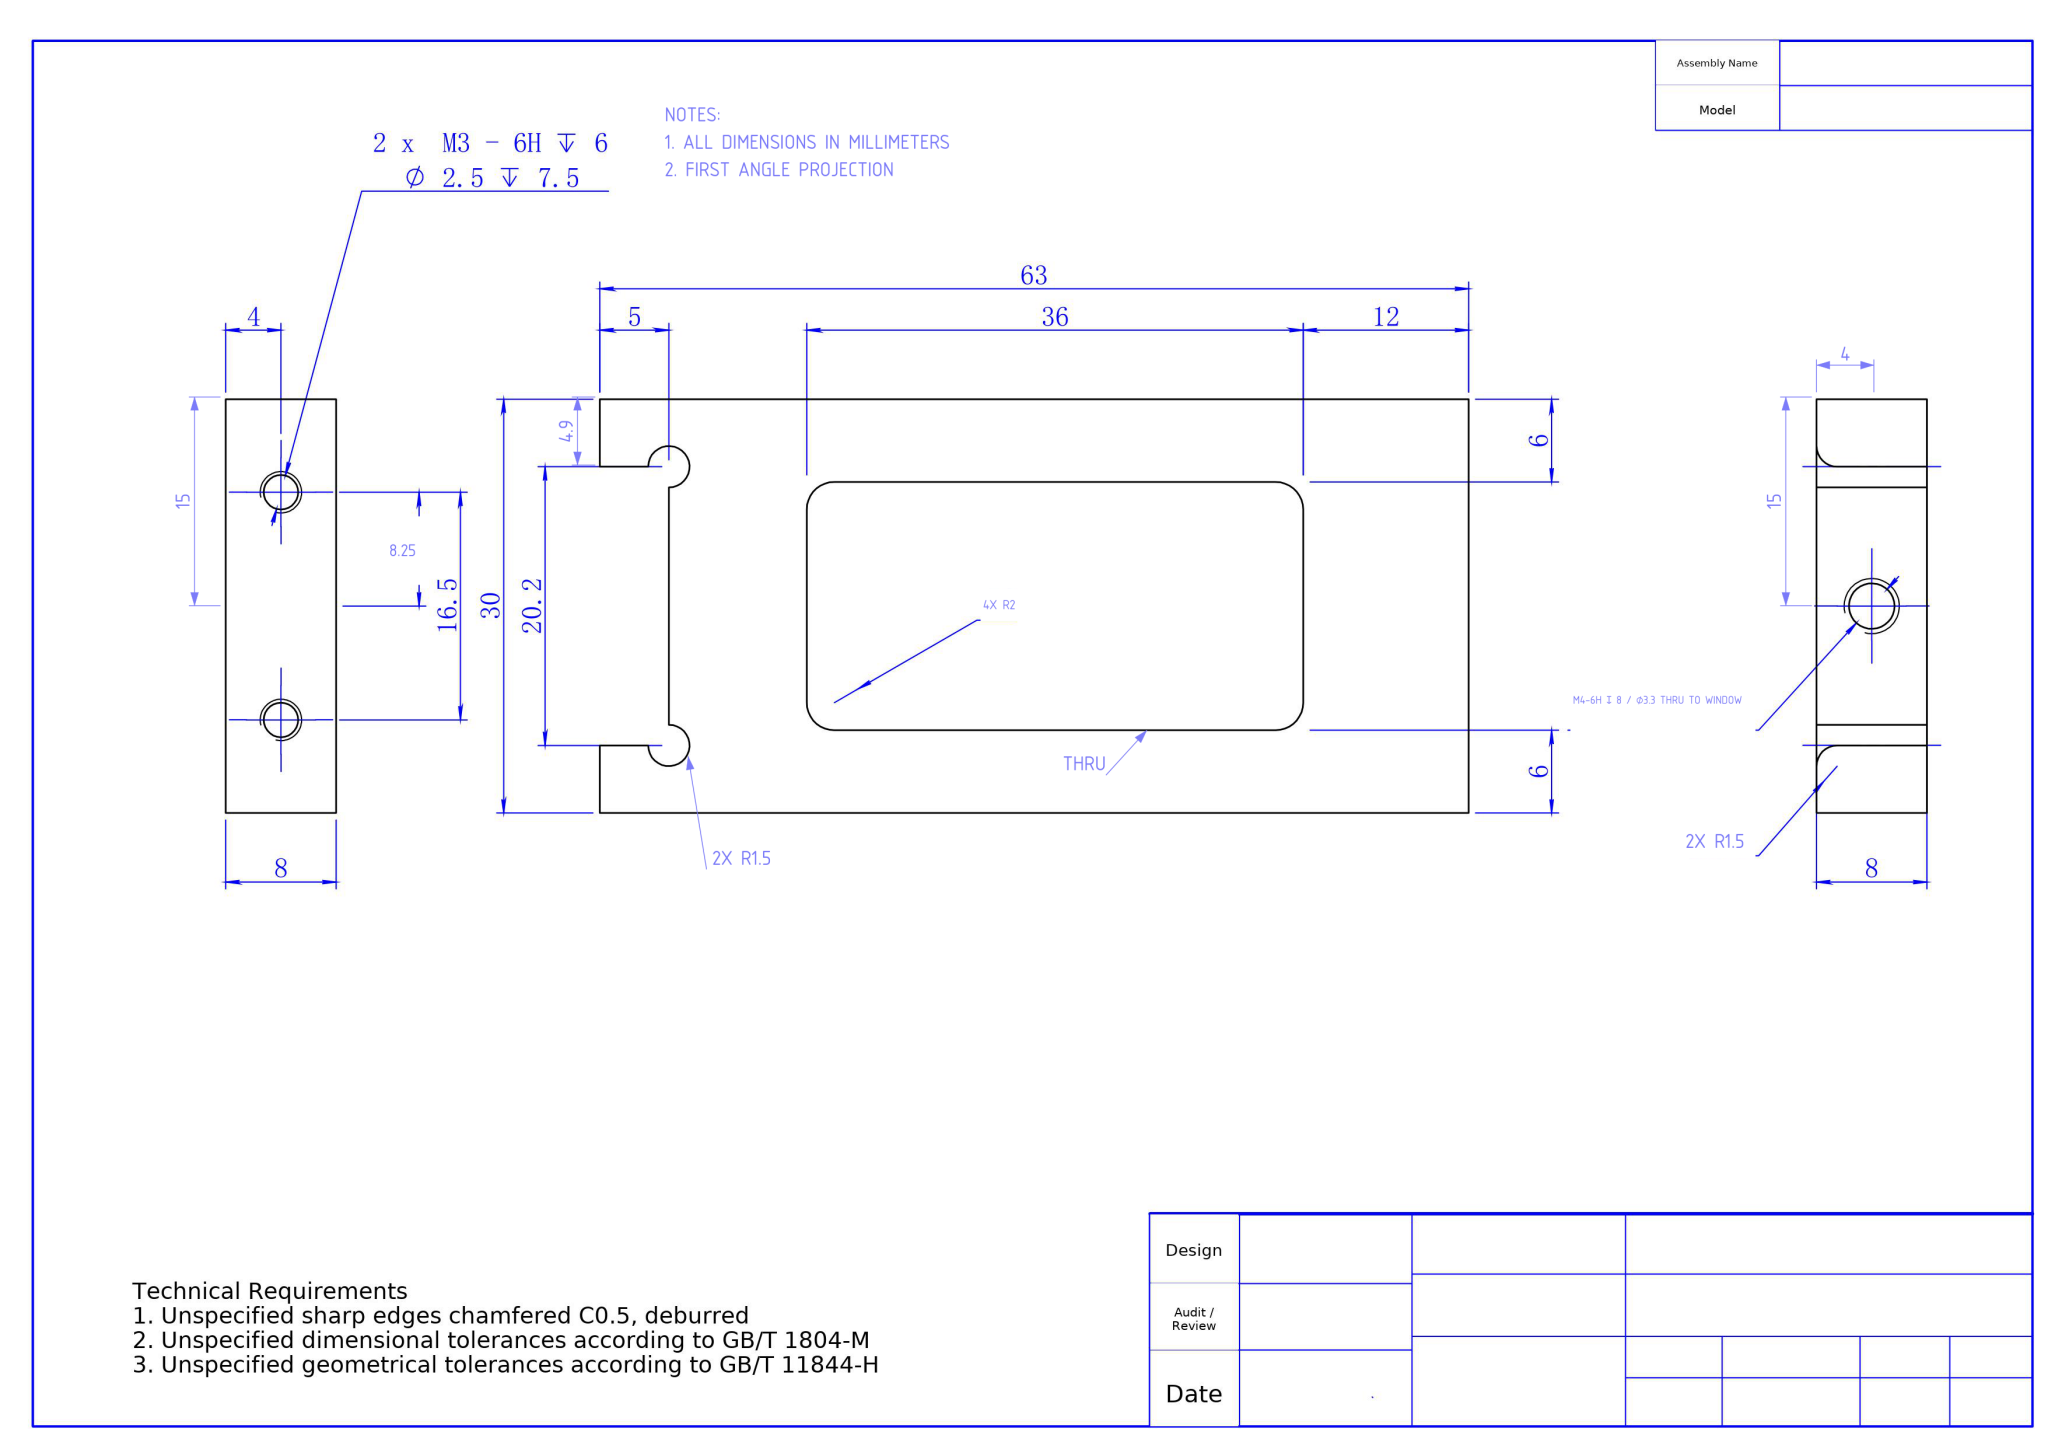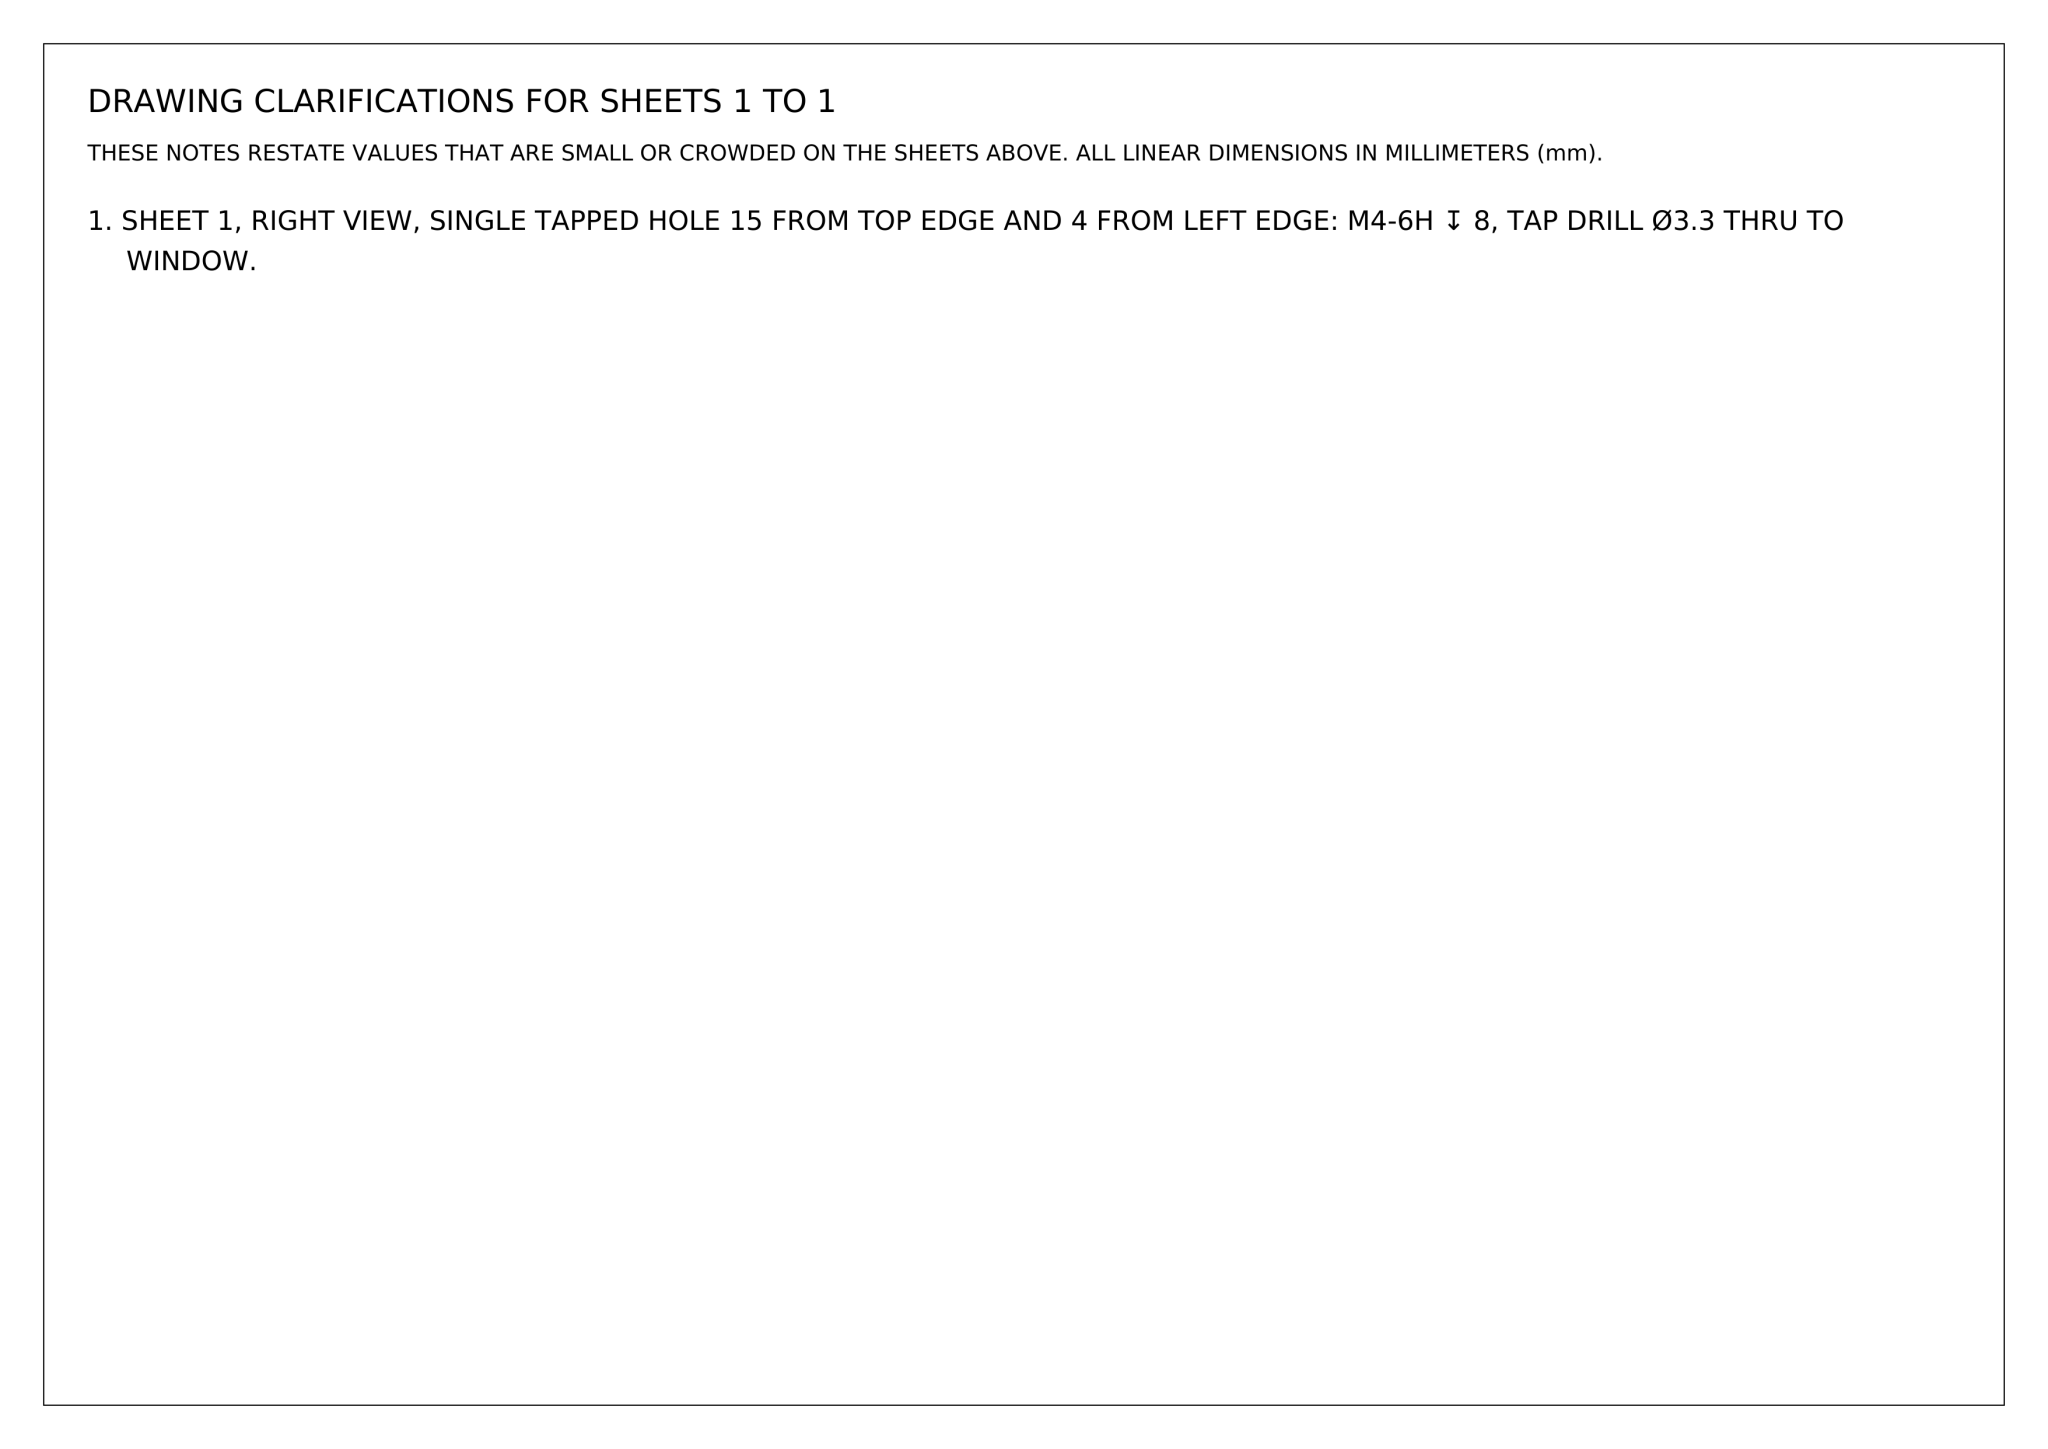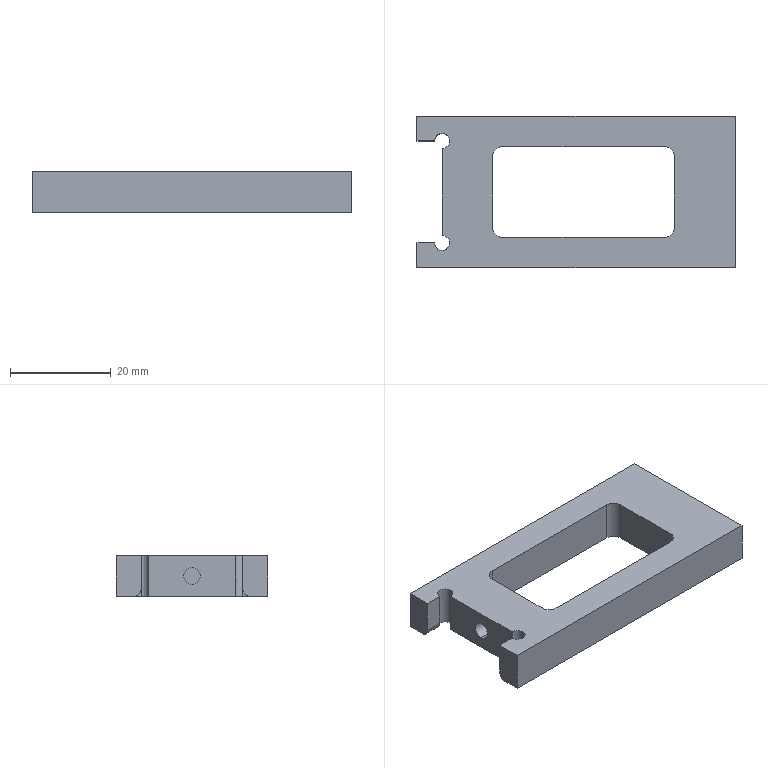Part | NX | mm | 1 solid | 34 faces | box 63 x 30 x 8 mm | volume 8906 mm3 | cylinder 16 | plane 14 | cone 4 | commonest cylinder face diameters 3 x6 2.5 x4 4 x4 3.3 x2